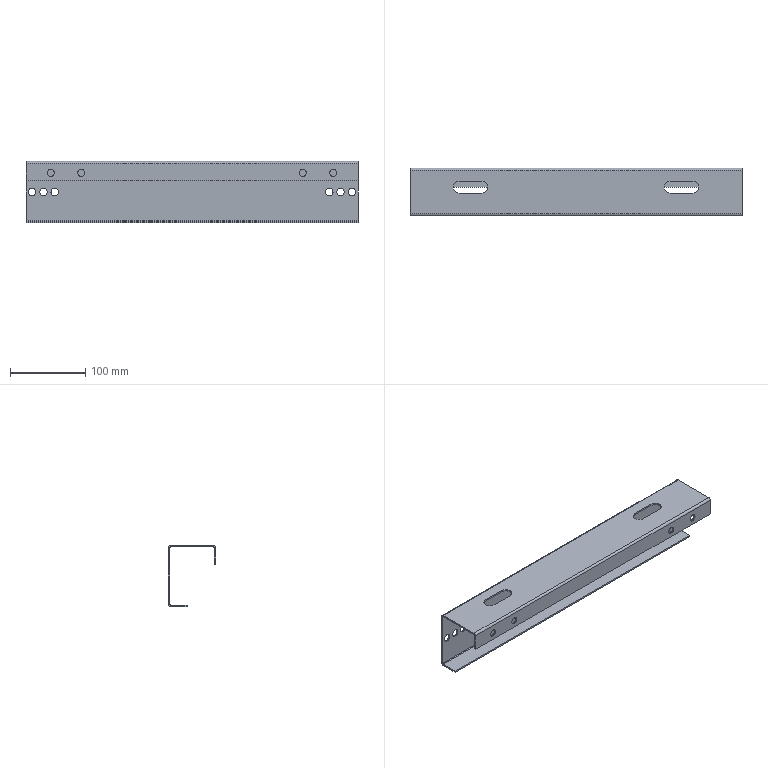Component | SolidWorks | 500CabinetWidthCrossbeamAssembly-1_500CabinetWidthCrossbeam-1 | 1 solid | 60 faces | volume 159274 mm3 | cylinder 32 | plane 28 | commonest cylinder face diameters 10 x12 9.2 x8 16 x6 5.473 x3 1.473 x3 | material Plain Carbon Steel